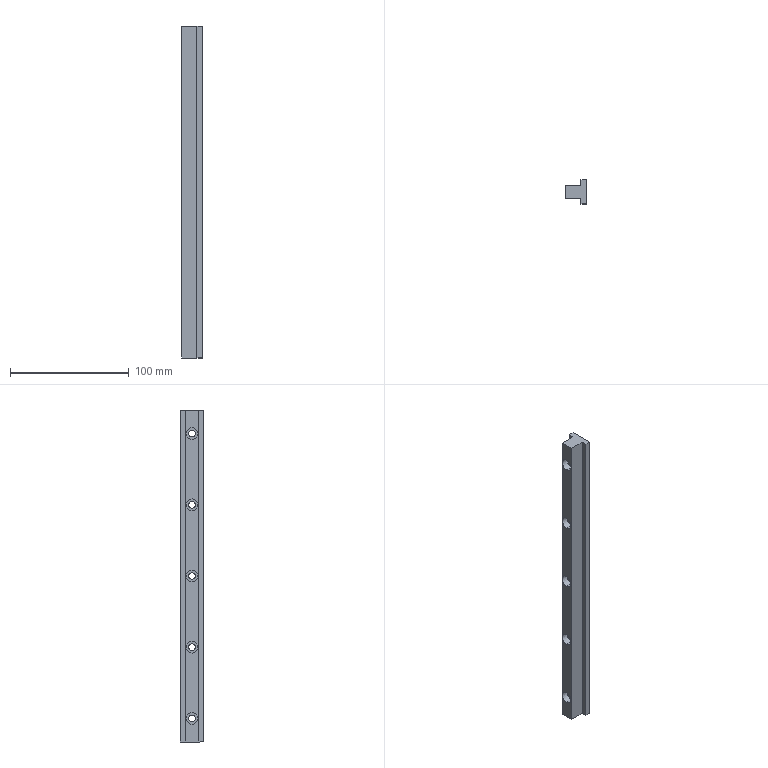Component | SolidWorks | GuideRailHGH-20CA-340-2 | 1 solid | 35 faces | box 17.5 x 20 x 280 mm | volume 61934 mm3 | cylinder 20 | plane 15 | commonest cylinder face diameters 5.5 x10 10 x10
build123d program:
from build123d import *

# Parameters (mm, degrees)
SKETCH1_W                                       = 20
SKETCH1_H                                       = 17.5
BOSS_EXTRUDE1_DEPTH                             = 280
SKETCH2_W                                       = 4.5
SKETCH2_H                                       = 12.9
CUT_EXTRUDE1_DEPTH                              = 280
M5_HEX_SOCKET_HEAD_CAP_SCREW_CBORE2_D           = 5.5
M5_HEX_SOCKET_HEAD_CAP_SCREW_CBORE2_CBORE_D     = 10
M5_HEX_SOCKET_HEAD_CAP_SCREW_CBORE2_CBORE_DEPTH = 5.4
LPATTERN1_COUNT                                 = 5
LPATTERN1_PITCH                                 = 60


with BuildPart() as part:
    # Sketch1 → Boss-Extrude1 (new body)
    with BuildSketch(Plane.XY):
        Rectangle(SKETCH1_W, SKETCH1_H)
    extrude(amount=BOSS_EXTRUDE1_DEPTH)

    # Sketch2 → Cut-Extrude1 (cut)
    with BuildSketch(Plane.XY.offset(280)):
        with Locations((-7.75, 2.3)):
            Rectangle(SKETCH2_W, SKETCH2_H)
        with Locations((7.75, 2.3)):
            Rectangle(SKETCH2_W, SKETCH2_H)
    extrude(amount=-CUT_EXTRUDE1_DEPTH, mode=Mode.SUBTRACT)

    # M5 Hex Socket Head Cap Screw CBORE2 (through all)
    with Locations(Plane(origin=(0, 8.75, 0), x_dir=(1, 0, 0), z_dir=(0, 1, 0))):
        with Locations((0, -260)):
            m5_hex_socket_head_cap_screw_cbore2 = CounterBoreHole(M5_HEX_SOCKET_HEAD_CAP_SCREW_CBORE2_D / 2, M5_HEX_SOCKET_HEAD_CAP_SCREW_CBORE2_CBORE_D / 2, M5_HEX_SOCKET_HEAD_CAP_SCREW_CBORE2_CBORE_DEPTH)

    # LPattern1: M5 Hex Socket Head Cap Screw CBORE2 ×5
    with Locations(*[(0, 0, -i * LPATTERN1_PITCH) for i in range(1, LPATTERN1_COUNT)]):
        add(m5_hex_socket_head_cap_screw_cbore2, mode=Mode.SUBTRACT)


solid = part.part

# Placed as in the assembly
solid = solid.moved(Location((1977.413, 3833.763, 939.241), (0, 0, 90)))
STEP:
#1=CARTESIAN_POINT('',(78.195,150.936,47.322));
#2=VERTEX_POINT('',#1);
#3=CARTESIAN_POINT('',(78.195,150.936,47.106));
#4=VERTEX_POINT('',#3);
#5=CARTESIAN_POINT('',(78.195,150.936,47.214));
#6=DIRECTION('',(-1.,-0.0001552,-0.));
#7=DIRECTION('',(0.,0.,-1.));
#8=AXIS2_PLACEMENT_3D('',#5,#6,#7);
#9=CIRCLE('',#8,0.1083);
#10=EDGE_CURVE('',#2,#4,#9,.T.);
#11=ORIENTED_EDGE('',*,*,#10,.F.);
#12=CARTESIAN_POINT('',(77.719,150.936,47.322));
#13=VERTEX_POINT('',#12);
#14=CARTESIAN_POINT('',(77.506,150.935,47.322));
#15=DIRECTION('',(-1.,-0.0001552,-0.));
#16=VECTOR('',#15,39.37);
#17=LINE('',#14,#16);
#18=EDGE_CURVE('',#2,#13,#17,.T.);
#19=ORIENTED_EDGE('',*,*,#18,.T.);
#20=CARTESIAN_POINT('',(77.719,150.936,47.106));
#21=VERTEX_POINT('',#20);
#22=CARTESIAN_POINT('',(77.719,150.936,47.214));
#23=DIRECTION('',(-1.,-0.0001552,-0.));
#24=DIRECTION('',(0.,0.,-1.));
#25=AXIS2_PLACEMENT_3D('',#22,#23,#24);
#26=CIRCLE('',#25,0.1083);
#27=EDGE_CURVE('',#13,#21,#26,.T.);
#28=ORIENTED_EDGE('',*,*,#27,.T.);
#29=CARTESIAN_POINT('',(77.506,150.935,47.106));
#30=DIRECTION('',(-1.,-0.0001552,-0.));
#31=VECTOR('',#30,39.37);
#32=LINE('',#29,#31);
#33=EDGE_CURVE('',#4,#21,#32,.T.);
#34=ORIENTED_EDGE('',*,*,#33,.F.);
#35=EDGE_LOOP('',(#11,#19,#28,#34));
#36=FACE_OUTER_BOUND('',#35,.T.);
#37=CARTESIAN_POINT('',(77.506,150.935,47.214));
#38=DIRECTION('',(-1.,-0.0001552,-0.));
#39=DIRECTION('',(0.,0.,-1.));
#40=AXIS2_PLACEMENT_3D('',#37,#38,#39);
#41=CYLINDRICAL_SURFACE('',#40,0.1083);
#42=ADVANCED_FACE('',(#36),#41,.F.);
#43=CARTESIAN_POINT('',(77.719,150.936,47.411));
#44=VERTEX_POINT('',#43);
#45=CARTESIAN_POINT('',(77.719,150.936,47.017));
#46=VERTEX_POINT('',#45);
#47=CARTESIAN_POINT('',(77.719,150.936,47.214));
#48=DIRECTION('',(-1.,-0.0001552,-0.));
#49=DIRECTION('',(0.,0.,-1.));
#50=AXIS2_PLACEMENT_3D('',#47,#48,#49);
#51=CIRCLE('',#50,0.1969);
#52=EDGE_CURVE('',#44,#46,#51,.T.);
#53=ORIENTED_EDGE('',*,*,#52,.F.);
#54=CARTESIAN_POINT('',(77.506,150.935,47.411));
#55=VERTEX_POINT('',#54);
#56=CARTESIAN_POINT('',(77.506,150.935,47.411));
#57=DIRECTION('',(-1.,-0.0001552,-0.));
#58=VECTOR('',#57,39.37);
#59=LINE('',#56,#58);
#60=EDGE_CURVE('',#44,#55,#59,.T.);
#61=ORIENTED_EDGE('',*,*,#60,.T.);
#62=CARTESIAN_POINT('',(77.506,150.935,47.017));
#63=VERTEX_POINT('',#62);
#64=CARTESIAN_POINT('',(77.506,150.935,47.214));
#65=DIRECTION('',(-1.,-0.0001552,-0.));
#66=DIRECTION('',(0.,0.,-1.));
#67=AXIS2_PLACEMENT_3D('',#64,#65,#66);
#68=CIRCLE('',#67,0.1969);
#69=EDGE_CURVE('',#55,#63,#68,.T.);
#70=ORIENTED_EDGE('',*,*,#69,.T.);
#71=CARTESIAN_POINT('',(77.506,150.935,47.017));
#72=DIRECTION('',(-1.,-0.0001552,-0.));
#73=VECTOR('',#72,39.37);
#74=LINE('',#71,#73);
#75=EDGE_CURVE('',#46,#63,#74,.T.);
#76=ORIENTED_EDGE('',*,*,#75,.F.);
#77=EDGE_LOOP('',(#53,#61,#70,#76));
#78=FACE_OUTER_BOUND('',#77,.T.);
#79=CARTESIAN_POINT('',(77.506,150.935,47.214));
#80=DIRECTION('',(-1.,-0.0001552,-0.));
#81=DIRECTION('',(0.,0.,-1.));
#82=AXIS2_PLACEMENT_3D('',#79,#80,#81);
#83=CYLINDRICAL_SURFACE('',#82,0.1969);
#84=ADVANCED_FACE('',(#78),#83,.F.);
#85=CARTESIAN_POINT('',(78.195,150.936,44.96));
#86=VERTEX_POINT('',#85);
#87=CARTESIAN_POINT('',(78.195,150.936,44.744));
#88=VERTEX_POINT('',#87);
#89=CARTESIAN_POINT('',(78.195,150.936,44.852));
#90=DIRECTION('',(-1.,-0.0001552,-0.));
#91=DIRECTION('',(0.,0.,-1.));
#92=AXIS2_PLACEMENT_3D('',#89,#90,#91);
#93=CIRCLE('',#92,0.1083);
#94=EDGE_CURVE('',#86,#88,#93,.T.);
#95=ORIENTED_EDGE('',*,*,#94,.F.);
#96=CARTESIAN_POINT('',(77.719,150.936,44.96));
#97=VERTEX_POINT('',#96);
#98=CARTESIAN_POINT('',(77.506,150.935,44.96));
#99=DIRECTION('',(-1.,-0.0001552,-0.));
#100=VECTOR('',#99,39.37);
#101=LINE('',#98,#100);
#102=EDGE_CURVE('',#86,#97,#101,.T.);
#103=ORIENTED_EDGE('',*,*,#102,.T.);
#104=CARTESIAN_POINT('',(77.719,150.936,44.744));
#105=VERTEX_POINT('',#104);
#106=CARTESIAN_POINT('',(77.719,150.936,44.852));
#107=DIRECTION('',(-1.,-0.0001552,-0.));
#108=DIRECTION('',(0.,0.,-1.));
#109=AXIS2_PLACEMENT_3D('',#106,#107,#108);
#110=CIRCLE('',#109,0.1083);
#111=EDGE_CURVE('',#97,#105,#110,.T.);
#112=ORIENTED_EDGE('',*,*,#111,.T.);
#113=CARTESIAN_POINT('',(77.506,150.935,44.744));
#114=DIRECTION('',(-1.,-0.0001552,-0.));
#115=VECTOR('',#114,39.37);
#116=LINE('',#113,#115);
#117=EDGE_CURVE('',#88,#105,#116,.T.);
#118=ORIENTED_EDGE('',*,*,#117,.F.);
#119=EDGE_LOOP('',(#95,#103,#112,#118));
#120=FACE_OUTER_BOUND('',#119,.T.);
#121=CARTESIAN_POINT('',(77.506,150.935,44.852));
#122=DIRECTION('',(-1.,-0.0001552,-0.));
#123=DIRECTION('',(0.,0.,-1.));
#124=AXIS2_PLACEMENT_3D('',#121,#122,#123);
#125=CYLINDRICAL_SURFACE('',#124,0.1083);
#126=ADVANCED_FACE('',(#120),#125,.F.);
#127=CARTESIAN_POINT('',(77.719,150.936,45.049));
#128=VERTEX_POINT('',#127);
#129=CARTESIAN_POINT('',(77.719,150.936,44.655));
#130=VERTEX_POINT('',#129);
#131=CARTESIAN_POINT('',(77.719,150.936,44.852));
#132=DIRECTION('',(-1.,-0.0001552,-0.));
#133=DIRECTION('',(0.,0.,-1.));
#134=AXIS2_PLACEMENT_3D('',#131,#132,#133);
#135=CIRCLE('',#134,0.1969);
#136=EDGE_CURVE('',#128,#130,#135,.T.);
#137=ORIENTED_EDGE('',*,*,#136,.F.);
#138=CARTESIAN_POINT('',(77.506,150.935,45.049));
#139=VERTEX_POINT('',#138);
#140=CARTESIAN_POINT('',(77.506,150.935,45.049));
#141=DIRECTION('',(-1.,-0.0001552,-0.));
#142=VECTOR('',#141,39.37);
#143=LINE('',#140,#142);
#144=EDGE_CURVE('',#128,#139,#143,.T.);
#145=ORIENTED_EDGE('',*,*,#144,.T.);
#146=CARTESIAN_POINT('',(77.506,150.935,44.655));
#147=VERTEX_POINT('',#146);
#148=CARTESIAN_POINT('',(77.506,150.935,44.852));
#149=DIRECTION('',(-1.,-0.0001552,-0.));
#150=DIRECTION('',(0.,0.,-1.));
#151=AXIS2_PLACEMENT_3D('',#148,#149,#150);
#152=CIRCLE('',#151,0.1969);
#153=EDGE_CURVE('',#139,#147,#152,.T.);
#154=ORIENTED_EDGE('',*,*,#153,.T.);
#155=CARTESIAN_POINT('',(77.506,150.935,44.655));
#156=DIRECTION('',(-1.,-0.0001552,-0.));
#157=VECTOR('',#156,39.37);
#158=LINE('',#155,#157);
#159=EDGE_CURVE('',#130,#147,#158,.T.);
#160=ORIENTED_EDGE('',*,*,#159,.F.);
#161=EDGE_LOOP('',(#137,#145,#154,#160));
#162=FACE_OUTER_BOUND('',#161,.T.);
#163=CARTESIAN_POINT('',(77.506,150.935,44.852));
#164=DIRECTION('',(-1.,-0.0001552,-0.));
#165=DIRECTION('',(0.,0.,-1.));
#166=AXIS2_PLACEMENT_3D('',#163,#164,#165);
#167=CYLINDRICAL_SURFACE('',#166,0.1969);
#168=ADVANCED_FACE('',(#162),#167,.F.);
#169=CARTESIAN_POINT('',(78.195,150.936,42.598));
#170=VERTEX_POINT('',#169);
#171=CARTESIAN_POINT('',(78.195,150.936,42.382));
#172=VERTEX_POINT('',#171);
#173=CARTESIAN_POINT('',(78.195,150.936,42.49));
#174=DIRECTION('',(-1.,-0.0001552,-0.));
#175=DIRECTION('',(0.,0.,-1.));
#176=AXIS2_PLACEMENT_3D('',#173,#174,#175);
#177=CIRCLE('',#176,0.1083);
#178=EDGE_CURVE('',#170,#172,#177,.T.);
#179=ORIENTED_EDGE('',*,*,#178,.F.);
#180=CARTESIAN_POINT('',(77.719,150.936,42.598));
#181=VERTEX_POINT('',#180);
#182=CARTESIAN_POINT('',(77.506,150.935,42.598));
#183=DIRECTION('',(-1.,-0.0001552,-0.));
#184=VECTOR('',#183,39.37);
#185=LINE('',#182,#184);
#186=EDGE_CURVE('',#170,#181,#185,.T.);
#187=ORIENTED_EDGE('',*,*,#186,.T.);
#188=CARTESIAN_POINT('',(77.719,150.936,42.382));
#189=VERTEX_POINT('',#188);
#190=CARTESIAN_POINT('',(77.719,150.936,42.49));
#191=DIRECTION('',(-1.,-0.0001552,-0.));
#192=DIRECTION('',(0.,0.,-1.));
#193=AXIS2_PLACEMENT_3D('',#190,#191,#192);
#194=CIRCLE('',#193,0.1083);
#195=EDGE_CURVE('',#181,#189,#194,.T.);
#196=ORIENTED_EDGE('',*,*,#195,.T.);
#197=CARTESIAN_POINT('',(77.506,150.935,42.382));
#198=DIRECTION('',(-1.,-0.0001552,-0.));
#199=VECTOR('',#198,39.37);
#200=LINE('',#197,#199);
#201=EDGE_CURVE('',#172,#189,#200,.T.);
#202=ORIENTED_EDGE('',*,*,#201,.F.);
#203=EDGE_LOOP('',(#179,#187,#196,#202));
#204=FACE_OUTER_BOUND('',#203,.T.);
#205=CARTESIAN_POINT('',(77.506,150.935,42.49));
#206=DIRECTION('',(-1.,-0.0001552,-0.));
#207=DIRECTION('',(0.,0.,-1.));
#208=AXIS2_PLACEMENT_3D('',#205,#206,#207);
#209=CYLINDRICAL_SURFACE('',#208,0.1083);
#210=ADVANCED_FACE('',(#204),#209,.F.);
#211=CARTESIAN_POINT('',(77.719,150.936,42.687));
#212=VERTEX_POINT('',#211);
#213=CARTESIAN_POINT('',(77.719,150.936,42.293));
#214=VERTEX_POINT('',#213);
#215=CARTESIAN_POINT('',(77.719,150.936,42.49));
#216=DIRECTION('',(-1.,-0.0001552,-0.));
#217=DIRECTION('',(0.,0.,-1.));
#218=AXIS2_PLACEMENT_3D('',#215,#216,#217);
#219=CIRCLE('',#218,0.1969);
#220=EDGE_CURVE('',#212,#214,#219,.T.);
#221=ORIENTED_EDGE('',*,*,#220,.F.);
#222=CARTESIAN_POINT('',(77.506,150.935,42.687));
#223=VERTEX_POINT('',#222);
#224=CARTESIAN_POINT('',(77.506,150.935,42.687));
#225=DIRECTION('',(-1.,-0.0001552,-0.));
#226=VECTOR('',#225,39.37);
#227=LINE('',#224,#226);
#228=EDGE_CURVE('',#212,#223,#227,.T.);
#229=ORIENTED_EDGE('',*,*,#228,.T.);
#230=CARTESIAN_POINT('',(77.506,150.935,42.293));
#231=VERTEX_POINT('',#230);
#232=CARTESIAN_POINT('',(77.506,150.935,42.49));
#233=DIRECTION('',(-1.,-0.0001552,-0.));
#234=DIRECTION('',(0.,0.,-1.));
#235=AXIS2_PLACEMENT_3D('',#232,#233,#234);
#236=CIRCLE('',#235,0.1969);
#237=EDGE_CURVE('',#223,#231,#236,.T.);
#238=ORIENTED_EDGE('',*,*,#237,.T.);
#239=CARTESIAN_POINT('',(77.506,150.935,42.293));
#240=DIRECTION('',(-1.,-0.0001552,-0.));
#241=VECTOR('',#240,39.37);
#242=LINE('',#239,#241);
#243=EDGE_CURVE('',#214,#231,#242,.T.);
#244=ORIENTED_EDGE('',*,*,#243,.F.);
#245=EDGE_LOOP('',(#221,#229,#238,#244));
#246=FACE_OUTER_BOUND('',#245,.T.);
#247=CARTESIAN_POINT('',(77.506,150.935,42.49));
#248=DIRECTION('',(-1.,-0.0001552,-0.));
#249=DIRECTION('',(0.,0.,-1.));
#250=AXIS2_PLACEMENT_3D('',#247,#248,#249);
#251=CYLINDRICAL_SURFACE('',#250,0.1969);
#252=ADVANCED_FACE('',(#246),#251,.F.);
#253=CARTESIAN_POINT('',(77.719,150.936,40.324));
#254=VERTEX_POINT('',#253);
#255=CARTESIAN_POINT('',(77.719,150.936,39.931));
#256=VERTEX_POINT('',#255);
#257=CARTESIAN_POINT('',(77.719,150.936,40.128));
#258=DIRECTION('',(-1.,-0.0001552,-0.));
#259=DIRECTION('',(0.,0.,-1.));
#260=AXIS2_PLACEMENT_3D('',#257,#258,#259);
#261=CIRCLE('',#260,0.1969);
#262=EDGE_CURVE('',#254,#256,#261,.T.);
#263=ORIENTED_EDGE('',*,*,#262,.F.);
#264=CARTESIAN_POINT('',(77.506,150.935,40.324));
#265=VERTEX_POINT('',#264);
#266=CARTESIAN_POINT('',(77.506,150.935,40.324));
#267=DIRECTION('',(-1.,-0.0001552,-0.));
#268=VECTOR('',#267,39.37);
#269=LINE('',#266,#268);
#270=EDGE_CURVE('',#254,#265,#269,.T.);
#271=ORIENTED_EDGE('',*,*,#270,.T.);
#272=CARTESIAN_POINT('',(77.506,150.935,39.931));
#273=VERTEX_POINT('',#272);
#274=CARTESIAN_POINT('',(77.506,150.935,40.128));
#275=DIRECTION('',(-1.,-0.0001552,-0.));
#276=DIRECTION('',(0.,0.,-1.));
#277=AXIS2_PLACEMENT_3D('',#274,#275,#276);
#278=CIRCLE('',#277,0.1969);
#279=EDGE_CURVE('',#265,#273,#278,.T.);
#280=ORIENTED_EDGE('',*,*,#279,.T.);
#281=CARTESIAN_POINT('',(77.506,150.935,39.931));
#282=DIRECTION('',(-1.,-0.0001552,-0.));
#283=VECTOR('',#282,39.37);
#284=LINE('',#281,#283);
#285=EDGE_CURVE('',#256,#273,#284,.T.);
#286=ORIENTED_EDGE('',*,*,#285,.F.);
#287=EDGE_LOOP('',(#263,#271,#280,#286));
#288=FACE_OUTER_BOUND('',#287,.T.);
#289=CARTESIAN_POINT('',(77.506,150.935,40.128));
#290=DIRECTION('',(-1.,-0.0001552,-0.));
#291=DIRECTION('',(0.,0.,-1.));
#292=AXIS2_PLACEMENT_3D('',#289,#290,#291);
#293=CYLINDRICAL_SURFACE('',#292,0.1969);
#294=ADVANCED_FACE('',(#288),#293,.F.);
#295=CARTESIAN_POINT('',(78.195,150.936,40.236));
#296=VERTEX_POINT('',#295);
#297=CARTESIAN_POINT('',(78.195,150.936,40.019));
#298=VERTEX_POINT('',#297);
#299=CARTESIAN_POINT('',(78.195,150.936,40.128));
#300=DIRECTION('',(-1.,-0.0001552,-0.));
#301=DIRECTION('',(0.,0.,-1.));
#302=AXIS2_PLACEMENT_3D('',#299,#300,#301);
#303=CIRCLE('',#302,0.1083);
#304=EDGE_CURVE('',#296,#298,#303,.T.);
#305=ORIENTED_EDGE('',*,*,#304,.F.);
#306=CARTESIAN_POINT('',(77.719,150.936,40.236));
#307=VERTEX_POINT('',#306);
#308=CARTESIAN_POINT('',(77.506,150.935,40.236));
#309=DIRECTION('',(-1.,-0.0001552,-0.));
#310=VECTOR('',#309,39.37);
#311=LINE('',#308,#310);
#312=EDGE_CURVE('',#296,#307,#311,.T.);
#313=ORIENTED_EDGE('',*,*,#312,.T.);
#314=CARTESIAN_POINT('',(77.719,150.936,40.019));
#315=VERTEX_POINT('',#314);
#316=CARTESIAN_POINT('',(77.719,150.936,40.128));
#317=DIRECTION('',(-1.,-0.0001552,-0.));
#318=DIRECTION('',(0.,0.,-1.));
#319=AXIS2_PLACEMENT_3D('',#316,#317,#318);
#320=CIRCLE('',#319,0.1083);
#321=EDGE_CURVE('',#307,#315,#320,.T.);
#322=ORIENTED_EDGE('',*,*,#321,.T.);
#323=CARTESIAN_POINT('',(77.506,150.935,40.019));
#324=DIRECTION('',(-1.,-0.0001552,-0.));
#325=VECTOR('',#324,39.37);
#326=LINE('',#323,#325);
#327=EDGE_CURVE('',#298,#315,#326,.T.);
#328=ORIENTED_EDGE('',*,*,#327,.F.);
#329=EDGE_LOOP('',(#305,#313,#322,#328));
#330=FACE_OUTER_BOUND('',#329,.T.);
#331=CARTESIAN_POINT('',(77.506,150.935,40.128));
#332=DIRECTION('',(-1.,-0.0001552,-0.));
#333=DIRECTION('',(0.,0.,-1.));
#334=AXIS2_PLACEMENT_3D('',#331,#332,#333);
#335=CYLINDRICAL_SURFACE('',#334,0.1083);
#336=ADVANCED_FACE('',(#330),#335,.F.);
#337=CARTESIAN_POINT('',(77.719,150.936,37.962));
#338=VERTEX_POINT('',#337);
#339=CARTESIAN_POINT('',(77.719,150.936,37.569));
#340=VERTEX_POINT('',#339);
#341=CARTESIAN_POINT('',(77.719,150.936,37.765));
#342=DIRECTION('',(-1.,-0.0001552,-0.));
#343=DIRECTION('',(0.,0.,-1.));
#344=AXIS2_PLACEMENT_3D('',#341,#342,#343);
#345=CIRCLE('',#344,0.1969);
#346=EDGE_CURVE('',#338,#340,#345,.T.);
#347=ORIENTED_EDGE('',*,*,#346,.F.);
#348=CARTESIAN_POINT('',(77.506,150.935,37.962));
#349=VERTEX_POINT('',#348);
#350=CARTESIAN_POINT('',(77.506,150.935,37.962));
#351=DIRECTION('',(-1.,-0.0001552,-0.));
#352=VECTOR('',#351,39.37);
#353=LINE('',#350,#352);
#354=EDGE_CURVE('',#338,#349,#353,.T.);
#355=ORIENTED_EDGE('',*,*,#354,.T.);
#356=CARTESIAN_POINT('',(77.506,150.935,37.569));
#357=VERTEX_POINT('',#356);
#358=CARTESIAN_POINT('',(77.506,150.935,37.765));
#359=DIRECTION('',(-1.,-0.0001552,-0.));
#360=DIRECTION('',(0.,0.,-1.));
#361=AXIS2_PLACEMENT_3D('',#358,#359,#360);
#362=CIRCLE('',#361,0.1969);
#363=EDGE_CURVE('',#349,#357,#362,.T.);
#364=ORIENTED_EDGE('',*,*,#363,.T.);
#365=CARTESIAN_POINT('',(77.506,150.935,37.569));
#366=DIRECTION('',(-1.,-0.0001552,-0.));
#367=VECTOR('',#366,39.37);
#368=LINE('',#365,#367);
#369=EDGE_CURVE('',#340,#357,#368,.T.);
#370=ORIENTED_EDGE('',*,*,#369,.F.);
#371=EDGE_LOOP('',(#347,#355,#364,#370));
#372=FACE_OUTER_BOUND('',#371,.T.);
#373=CARTESIAN_POINT('',(77.506,150.935,37.765));
#374=DIRECTION('',(-1.,-0.0001552,-0.));
#375=DIRECTION('',(0.,0.,-1.));
#376=AXIS2_PLACEMENT_3D('',#373,#374,#375);
#377=CYLINDRICAL_SURFACE('',#376,0.1969);
#378=ADVANCED_FACE('',(#372),#377,.F.);
#379=CARTESIAN_POINT('',(78.195,150.936,37.874));
#380=VERTEX_POINT('',#379);
#381=CARTESIAN_POINT('',(78.195,150.936,37.657));
#382=VERTEX_POINT('',#381);
#383=CARTESIAN_POINT('',(78.195,150.936,37.765));
#384=DIRECTION('',(-1.,-0.0001552,-0.));
#385=DIRECTION('',(0.,0.,-1.));
#386=AXIS2_PLACEMENT_3D('',#383,#384,#385);
#387=CIRCLE('',#386,0.1083);
#388=EDGE_CURVE('',#380,#382,#387,.T.);
#389=ORIENTED_EDGE('',*,*,#388,.F.);
#390=CARTESIAN_POINT('',(77.719,150.936,37.874));
#391=VERTEX_POINT('',#390);
#392=CARTESIAN_POINT('',(77.506,150.935,37.874));
#393=DIRECTION('',(-1.,-0.0001552,-0.));
#394=VECTOR('',#393,39.37);
#395=LINE('',#392,#394);
#396=EDGE_CURVE('',#380,#391,#395,.T.);
#397=ORIENTED_EDGE('',*,*,#396,.T.);
#398=CARTESIAN_POINT('',(77.719,150.936,37.657));
#399=VERTEX_POINT('',#398);
#400=CARTESIAN_POINT('',(77.719,150.936,37.765));
#401=DIRECTION('',(-1.,-0.0001552,-0.));
#402=DIRECTION('',(0.,0.,-1.));
#403=AXIS2_PLACEMENT_3D('',#400,#401,#402);
#404=CIRCLE('',#403,0.1083);
#405=EDGE_CURVE('',#391,#399,#404,.T.);
#406=ORIENTED_EDGE('',*,*,#405,.T.);
#407=CARTESIAN_POINT('',(77.506,150.935,37.657));
#408=DIRECTION('',(-1.,-0.0001552,-0.));
#409=VECTOR('',#408,39.37);
#410=LINE('',#407,#409);
#411=EDGE_CURVE('',#382,#399,#410,.T.);
#412=ORIENTED_EDGE('',*,*,#411,.F.);
#413=EDGE_LOOP('',(#389,#397,#406,#412));
#414=FACE_OUTER_BOUND('',#413,.T.);
#415=CARTESIAN_POINT('',(77.506,150.935,37.765));
#416=DIRECTION('',(-1.,-0.0001552,-0.));
#417=DIRECTION('',(0.,0.,-1.));
#418=AXIS2_PLACEMENT_3D('',#415,#416,#417);
#419=CYLINDRICAL_SURFACE('',#418,0.1083);
#420=ADVANCED_FACE('',(#414),#419,.F.);
#421=CARTESIAN_POINT('',(78.014,151.329,36.978));
#422=VERTEX_POINT('',#421);
#423=CARTESIAN_POINT('',(78.195,151.329,36.978));
#424=VERTEX_POINT('',#423);
#425=CARTESIAN_POINT('',(78.195,151.329,36.978));
#426=DIRECTION('',(1.,0.0001552,0.));
#427=VECTOR('',#426,39.37);
#428=LINE('',#425,#427);
#429=EDGE_CURVE('',#422,#424,#428,.T.);
#430=ORIENTED_EDGE('',*,*,#429,.F.);
#431=CARTESIAN_POINT('',(78.014,151.329,48.002));
#432=VERTEX_POINT('',#431);
#433=CARTESIAN_POINT('',(78.014,151.329,48.54));
#434=DIRECTION('',(0.,-0.,-1.));
#435=VECTOR('',#434,39.37);
#436=LINE('',#433,#435);
#437=EDGE_CURVE('',#432,#422,#436,.T.);
#438=ORIENTED_EDGE('',*,*,#437,.F.);
#439=CARTESIAN_POINT('',(78.195,151.329,48.002));
#440=VERTEX_POINT('',#439);
#441=CARTESIAN_POINT('',(78.195,151.329,48.002));
#442=DIRECTION('',(1.,0.0001552,0.));
#443=VECTOR('',#442,39.37);
#444=LINE('',#441,#443);
#445=EDGE_CURVE('',#432,#440,#444,.T.);
#446=ORIENTED_EDGE('',*,*,#445,.T.);
#447=CARTESIAN_POINT('',(78.195,151.329,36.978));
#448=DIRECTION('',(-0.,0.,1.));
#449=VECTOR('',#448,39.37);
#450=LINE('',#447,#449);
#451=EDGE_CURVE('',#424,#440,#450,.T.);
#452=ORIENTED_EDGE('',*,*,#451,.F.);
#453=EDGE_LOOP('',(#430,#438,#446,#452));
#454=FACE_OUTER_BOUND('',#453,.T.);
#455=CARTESIAN_POINT('',(78.195,151.329,36.978));
#456=DIRECTION('',(0.0001552,-1.,0.));
#457=DIRECTION('',(-0.,0.,1.));
#458=AXIS2_PLACEMENT_3D('',#455,#456,#457);
#459=PLANE('',#458);
#460=ADVANCED_FACE('',(#454),#459,.F.);
#461=CARTESIAN_POINT('',(78.195,150.936,40.128));
#462=DIRECTION('',(-1.,-0.0001552,-0.));
#463=DIRECTION('',(0.,0.,-1.));
#464=AXIS2_PLACEMENT_3D('',#461,#462,#463);
#465=CIRCLE('',#464,0.1083);
#466=EDGE_CURVE('',#298,#296,#465,.T.);
#467=ORIENTED_EDGE('',*,*,#466,.T.);
#468=ORIENTED_EDGE('',*,*,#304,.T.);
#469=EDGE_LOOP('',(#467,#468));
#470=FACE_BOUND('',#469,.T.);
#471=CARTESIAN_POINT('',(78.195,150.936,37.765));
#472=DIRECTION('',(-1.,-0.0001552,-0.));
#473=DIRECTION('',(0.,0.,-1.));
#474=AXIS2_PLACEMENT_3D('',#471,#472,#473);
#475=CIRCLE('',#474,0.1083);
#476=EDGE_CURVE('',#382,#380,#475,.T.);
#477=ORIENTED_EDGE('',*,*,#476,.T.);
#478=ORIENTED_EDGE('',*,*,#388,.T.);
#479=EDGE_LOOP('',(#477,#478));
#480=FACE_BOUND('',#479,.T.);
#481=CARTESIAN_POINT('',(78.195,150.542,48.002));
#482=VERTEX_POINT('',#481);
#483=CARTESIAN_POINT('',(78.195,150.542,48.002));
#484=DIRECTION('',(0.0001552,-1.,0.));
#485=VECTOR('',#484,39.37);
#486=LINE('',#483,#485);
#487=EDGE_CURVE('',#440,#482,#486,.T.);
#488=ORIENTED_EDGE('',*,*,#487,.T.);
#489=CARTESIAN_POINT('',(78.195,150.542,36.978));
#490=VERTEX_POINT('',#489);
#491=CARTESIAN_POINT('',(78.195,150.542,36.978));
#492=DIRECTION('',(-0.,0.,1.));
#493=VECTOR('',#492,39.37);
#494=LINE('',#491,#493);
#495=EDGE_CURVE('',#490,#482,#494,.T.);
#496=ORIENTED_EDGE('',*,*,#495,.F.);
#497=CARTESIAN_POINT('',(78.195,150.542,36.978));
#498=DIRECTION('',(0.0001552,-1.,0.));
#499=VECTOR('',#498,39.37);
#500=LINE('',#497,#499);
#501=EDGE_CURVE('',#424,#490,#500,.T.);
#502=ORIENTED_EDGE('',*,*,#501,.F.);
#503=ORIENTED_EDGE('',*,*,#451,.T.);
#504=EDGE_LOOP('',(#488,#496,#502,#503));
#505=FACE_OUTER_BOUND('',#504,.T.);
#506=CARTESIAN_POINT('',(78.195,150.936,42.49));
#507=DIRECTION('',(-1.,-0.0001552,-0.));
#508=DIRECTION('',(0.,0.,-1.));
#509=AXIS2_PLACEMENT_3D('',#506,#507,#508);
#510=CIRCLE('',#509,0.1083);
#511=EDGE_CURVE('',#172,#170,#510,.T.);
#512=ORIENTED_EDGE('',*,*,#511,.T.);
#513=ORIENTED_EDGE('',*,*,#178,.T.);
#514=EDGE_LOOP('',(#512,#513));
#515=FACE_BOUND('',#514,.T.);
#516=CARTESIAN_POINT('',(78.195,150.936,44.852));
#517=DIRECTION('',(-1.,-0.0001552,-0.));
#518=DIRECTION('',(0.,0.,-1.));
#519=AXIS2_PLACEMENT_3D('',#516,#517,#518);
#520=CIRCLE('',#519,0.1083);
#521=EDGE_CURVE('',#88,#86,#520,.T.);
#522=ORIENTED_EDGE('',*,*,#521,.T.);
#523=ORIENTED_EDGE('',*,*,#94,.T.);
#524=EDGE_LOOP('',(#522,#523));
#525=FACE_BOUND('',#524,.T.);
#526=CARTESIAN_POINT('',(78.195,150.936,47.214));
#527=DIRECTION('',(-1.,-0.0001552,-0.));
#528=DIRECTION('',(0.,0.,-1.));
#529=AXIS2_PLACEMENT_3D('',#526,#527,#528);
#530=CIRCLE('',#529,0.1083);
#531=EDGE_CURVE('',#4,#2,#530,.T.);
#532=ORIENTED_EDGE('',*,*,#531,.T.);
#533=ORIENTED_EDGE('',*,*,#10,.T.);
#534=EDGE_LOOP('',(#532,#533));
#535=FACE_BOUND('',#534,.T.);
#536=CARTESIAN_POINT('',(78.195,150.542,36.978));
#537=DIRECTION('',(-1.,-0.0001552,-0.));
#538=DIRECTION('',(-0.0001552,1.,-0.));
#539=AXIS2_PLACEMENT_3D('',#536,#537,#538);
#540=PLANE('',#539);
#541=ADVANCED_FACE('',(#470,#480,#505,#515,#525,#535),#540,.F.);
#542=CARTESIAN_POINT('',(78.014,150.542,48.002));
#543=VERTEX_POINT('',#542);
#544=CARTESIAN_POINT('',(78.195,150.542,48.002));
#545=DIRECTION('',(-1.,-0.0001552,-0.));
#546=VECTOR('',#545,39.37);
#547=LINE('',#544,#546);
#548=EDGE_CURVE('',#482,#543,#547,.T.);
#549=ORIENTED_EDGE('',*,*,#548,.T.);
#550=CARTESIAN_POINT('',(78.014,150.542,36.978));
#551=VERTEX_POINT('',#550);
#552=CARTESIAN_POINT('',(78.014,150.542,48.54));
#553=DIRECTION('',(0.,-0.,-1.));
#554=VECTOR('',#553,39.37);
#555=LINE('',#552,#554);
#556=EDGE_CURVE('',#543,#551,#555,.T.);
#557=ORIENTED_EDGE('',*,*,#556,.T.);
#558=CARTESIAN_POINT('',(78.195,150.542,36.978));
#559=DIRECTION('',(-1.,-0.0001552,-0.));
#560=VECTOR('',#559,39.37);
#561=LINE('',#558,#560);
#562=EDGE_CURVE('',#490,#551,#561,.T.);
#563=ORIENTED_EDGE('',*,*,#562,.F.);
#564=ORIENTED_EDGE('',*,*,#495,.T.);
#565=EDGE_LOOP('',(#549,#557,#563,#564));
#566=FACE_OUTER_BOUND('',#565,.T.);
#567=CARTESIAN_POINT('',(78.195,150.542,36.978));
#568=DIRECTION('',(-0.0001552,1.,-0.));
#569=DIRECTION('',(0.,-0.,-1.));
#570=AXIS2_PLACEMENT_3D('',#567,#568,#569);
#571=PLANE('',#570);
#572=ADVANCED_FACE('',(#566),#571,.F.);
#573=CARTESIAN_POINT('',(77.506,150.935,40.128));
#574=DIRECTION('',(-1.,-0.0001552,-0.));
#575=DIRECTION('',(0.,0.,-1.));
#576=AXIS2_PLACEMENT_3D('',#573,#574,#575);
#577=CIRCLE('',#576,0.1969);
#578=EDGE_CURVE('',#273,#265,#577,.T.);
#579=ORIENTED_EDGE('',*,*,#578,.F.);
#580=ORIENTED_EDGE('',*,*,#279,.F.);
#581=EDGE_LOOP('',(#579,#580));
#582=FACE_BOUND('',#581,.T.);
#583=CARTESIAN_POINT('',(77.506,150.935,37.765));
#584=DIRECTION('',(-1.,-0.0001552,-0.));
#585=DIRECTION('',(0.,0.,-1.));
#586=AXIS2_PLACEMENT_3D('',#583,#584,#585);
#587=CIRCLE('',#586,0.1969);
#588=EDGE_CURVE('',#357,#349,#587,.T.);
#589=ORIENTED_EDGE('',*,*,#588,.F.);
#590=ORIENTED_EDGE('',*,*,#363,.F.);
#591=EDGE_LOOP('',(#589,#590));
#592=FACE_BOUND('',#591,.T.);
#593=CARTESIAN_POINT('',(77.506,150.719,36.978));
#594=VERTEX_POINT('',#593);
#595=CARTESIAN_POINT('',(77.506,151.152,36.978));
#596=VERTEX_POINT('',#595);
#597=CARTESIAN_POINT('',(77.506,150.542,36.978));
#598=DIRECTION('',(-0.0001552,1.,-0.));
#599=VECTOR('',#598,39.37);
#600=LINE('',#597,#599);
#601=EDGE_CURVE('',#594,#596,#600,.T.);
#602=ORIENTED_EDGE('',*,*,#601,.F.);
#603=CARTESIAN_POINT('',(77.506,150.719,48.002));
#604=VERTEX_POINT('',#603);
#605=CARTESIAN_POINT('',(77.506,150.719,48.54));
#606=DIRECTION('',(0.,-0.,-1.));
#607=VECTOR('',#606,39.37);
#608=LINE('',#605,#607);
#609=EDGE_CURVE('',#604,#594,#608,.T.);
#610=ORIENTED_EDGE('',*,*,#609,.F.);
#611=CARTESIAN_POINT('',(77.506,151.152,48.002));
#612=VERTEX_POINT('',#611);
#613=CARTESIAN_POINT('',(77.506,150.542,48.002));
#614=DIRECTION('',(-0.0001552,1.,-0.));
#615=VECTOR('',#614,39.37);
#616=LINE('',#613,#615);
#617=EDGE_CURVE('',#604,#612,#616,.T.);
#618=ORIENTED_EDGE('',*,*,#617,.T.);
#619=CARTESIAN_POINT('',(77.506,151.152,48.54));
#620=DIRECTION('',(0.,-0.,-1.));
#621=VECTOR('',#620,39.37);
#622=LINE('',#619,#621);
#623=EDGE_CURVE('',#612,#596,#622,.T.);
#624=ORIENTED_EDGE('',*,*,#623,.T.);
#625=EDGE_LOOP('',(#602,#610,#618,#624));
#626=FACE_OUTER_BOUND('',#625,.T.);
#627=CARTESIAN_POINT('',(77.506,150.935,42.49));
#628=DIRECTION('',(-1.,-0.0001552,-0.));
#629=DIRECTION('',(0.,0.,-1.));
#630=AXIS2_PLACEMENT_3D('',#627,#628,#629);
#631=CIRCLE('',#630,0.1969);
#632=EDGE_CURVE('',#231,#223,#631,.T.);
#633=ORIENTED_EDGE('',*,*,#632,.F.);
#634=ORIENTED_EDGE('',*,*,#237,.F.);
#635=EDGE_LOOP('',(#633,#634));
#636=FACE_BOUND('',#635,.T.);
#637=CARTESIAN_POINT('',(77.506,150.935,44.852));
#638=DIRECTION('',(-1.,-0.0001552,-0.));
#639=DIRECTION('',(0.,0.,-1.));
#640=AXIS2_PLACEMENT_3D('',#637,#638,#639);
#641=CIRCLE('',#640,0.1969);
#642=EDGE_CURVE('',#147,#139,#641,.T.);
#643=ORIENTED_EDGE('',*,*,#642,.F.);
#644=ORIENTED_EDGE('',*,*,#153,.F.);
#645=EDGE_LOOP('',(#643,#644));
#646=FACE_BOUND('',#645,.T.);
#647=CARTESIAN_POINT('',(77.506,150.935,47.214));
#648=DIRECTION('',(-1.,-0.0001552,-0.));
#649=DIRECTION('',(0.,0.,-1.));
#650=AXIS2_PLACEMENT_3D('',#647,#648,#649);
#651=CIRCLE('',#650,0.1969);
#652=EDGE_CURVE('',#63,#55,#651,.T.);
#653=ORIENTED_EDGE('',*,*,#652,.F.);
#654=ORIENTED_EDGE('',*,*,#69,.F.);
#655=EDGE_LOOP('',(#653,#654));
#656=FACE_BOUND('',#655,.T.);
#657=CARTESIAN_POINT('',(77.506,150.542,36.978));
#658=DIRECTION('',(1.,0.0001552,0.));
#659=DIRECTION('',(0.0001552,-1.,0.));
#660=AXIS2_PLACEMENT_3D('',#657,#658,#659);
#661=PLANE('',#660);
#662=ADVANCED_FACE('',(#582,#592,#626,#636,#646,#656),#661,.F.);
#663=CARTESIAN_POINT('',(78.014,150.719,36.978));
#664=VERTEX_POINT('',#663);
#665=CARTESIAN_POINT('',(78.014,150.542,36.978));
#666=DIRECTION('',(0.0001552,-1.,0.));
#667=VECTOR('',#666,39.37);
#668=LINE('',#665,#667);
#669=EDGE_CURVE('',#664,#551,#668,.T.);
#670=ORIENTED_EDGE('',*,*,#669,.F.);
#671=CARTESIAN_POINT('',(78.014,150.719,36.978));
#672=DIRECTION('',(1.,0.0001552,0.));
#673=VECTOR('',#672,39.37);
#674=LINE('',#671,#673);
#675=EDGE_CURVE('',#594,#664,#674,.T.);
#676=ORIENTED_EDGE('',*,*,#675,.F.);
#677=ORIENTED_EDGE('',*,*,#601,.T.);
#678=CARTESIAN_POINT('',(78.014,151.152,36.978));
#679=VERTEX_POINT('',#678);
#680=CARTESIAN_POINT('',(78.014,151.152,36.978));
#681=DIRECTION('',(-1.,-0.0001552,-0.));
#682=VECTOR('',#681,39.37);
#683=LINE('',#680,#682);
#684=EDGE_CURVE('',#679,#596,#683,.T.);
#685=ORIENTED_EDGE('',*,*,#684,.F.);
#686=CARTESIAN_POINT('',(78.014,151.329,36.978));
#687=DIRECTION('',(0.0001552,-1.,0.));
#688=VECTOR('',#687,39.37);
#689=LINE('',#686,#688);
#690=EDGE_CURVE('',#422,#679,#689,.T.);
#691=ORIENTED_EDGE('',*,*,#690,.F.);
#692=ORIENTED_EDGE('',*,*,#429,.T.);
#693=ORIENTED_EDGE('',*,*,#501,.T.);
#694=ORIENTED_EDGE('',*,*,#562,.T.);
#695=EDGE_LOOP('',(#670,#676,#677,#685,#691,#692,#693,#694));
#696=FACE_OUTER_BOUND('',#695,.T.);
#697=CARTESIAN_POINT('',(77.851,150.936,36.978));
#698=DIRECTION('',(0.,-0.,-1.));
#699=DIRECTION('',(0.0001552,-1.,0.));
#700=AXIS2_PLACEMENT_3D('',#697,#698,#699);
#701=PLANE('',#700);
#702=ADVANCED_FACE('',(#696),#701,.T.);
#703=CARTESIAN_POINT('',(78.014,150.719,48.002));
#704=VERTEX_POINT('',#703);
#705=CARTESIAN_POINT('',(78.014,150.719,48.002));
#706=DIRECTION('',(-1.,-0.0001552,-0.));
#707=VECTOR('',#706,39.37);
#708=LINE('',#705,#707);
#709=EDGE_CURVE('',#704,#604,#708,.T.);
#710=ORIENTED_EDGE('',*,*,#709,.F.);
#711=CARTESIAN_POINT('',(78.014,150.542,48.002));
#712=DIRECTION('',(-0.0001552,1.,-0.));
#713=VECTOR('',#712,39.37);
#714=LINE('',#711,#713);
#715=EDGE_CURVE('',#543,#704,#714,.T.);
#716=ORIENTED_EDGE('',*,*,#715,.F.);
#717=ORIENTED_EDGE('',*,*,#548,.F.);
#718=ORIENTED_EDGE('',*,*,#487,.F.);
#719=ORIENTED_EDGE('',*,*,#445,.F.);
#720=CARTESIAN_POINT('',(78.014,151.152,48.002));
#721=VERTEX_POINT('',#720);
#722=CARTESIAN_POINT('',(78.014,151.329,48.002));
#723=DIRECTION('',(-0.0001552,1.,-0.));
#724=VECTOR('',#723,39.37);
#725=LINE('',#722,#724);
#726=EDGE_CURVE('',#721,#432,#725,.T.);
#727=ORIENTED_EDGE('',*,*,#726,.F.);
#728=CARTESIAN_POINT('',(78.014,151.152,48.002));
#729=DIRECTION('',(1.,0.0001552,0.));
#730=VECTOR('',#729,39.37);
#731=LINE('',#728,#730);
#732=EDGE_CURVE('',#612,#721,#731,.T.);
#733=ORIENTED_EDGE('',*,*,#732,.F.);
#734=ORIENTED_EDGE('',*,*,#617,.F.);
#735=EDGE_LOOP('',(#710,#716,#717,#718,#719,#727,#733,#734));
#736=FACE_OUTER_BOUND('',#735,.T.);
#737=CARTESIAN_POINT('',(77.851,150.936,48.002));
#738=DIRECTION('',(0.,-0.,-1.));
#739=DIRECTION('',(0.0001552,-1.,0.));
#740=AXIS2_PLACEMENT_3D('',#737,#738,#739);
#741=PLANE('',#740);
#742=ADVANCED_FACE('',(#736),#741,.F.);
#743=ORIENTED_EDGE('',*,*,#732,.T.);
#744=CARTESIAN_POINT('',(78.014,151.152,48.54));
#745=DIRECTION('',(0.,-0.,-1.));
#746=VECTOR('',#745,39.37);
#747=LINE('',#744,#746);
#748=EDGE_CURVE('',#721,#679,#747,.T.);
#749=ORIENTED_EDGE('',*,*,#748,.T.);
#750=ORIENTED_EDGE('',*,*,#684,.T.);
#751=ORIENTED_EDGE('',*,*,#623,.F.);
#752=EDGE_LOOP('',(#743,#749,#750,#751));
#753=FACE_OUTER_BOUND('',#752,.T.);
#754=CARTESIAN_POINT('',(78.014,151.152,48.54));
#755=DIRECTION('',(0.0001552,-1.,0.));
#756=DIRECTION('',(-0.,0.,1.));
#757=AXIS2_PLACEMENT_3D('',#754,#755,#756);
#758=PLANE('',#757);
#759=ADVANCED_FACE('',(#753),#758,.F.);
#760=ORIENTED_EDGE('',*,*,#726,.T.);
#761=ORIENTED_EDGE('',*,*,#437,.T.);
#762=ORIENTED_EDGE('',*,*,#690,.T.);
#763=ORIENTED_EDGE('',*,*,#748,.F.);
#764=EDGE_LOOP('',(#760,#761,#762,#763));
#765=FACE_OUTER_BOUND('',#764,.T.);
#766=CARTESIAN_POINT('',(78.014,151.329,48.54));
#767=DIRECTION('',(1.,0.0001552,0.));
#768=DIRECTION('',(-0.,0.,1.));
#769=AXIS2_PLACEMENT_3D('',#766,#767,#768);
#770=PLANE('',#769);
#771=ADVANCED_FACE('',(#765),#770,.F.);
#772=ORIENTED_EDGE('',*,*,#715,.T.);
#773=CARTESIAN_POINT('',(78.014,150.719,48.54));
#774=DIRECTION('',(0.,-0.,-1.));
#775=VECTOR('',#774,39.37);
#776=LINE('',#773,#775);
#777=EDGE_CURVE('',#704,#664,#776,.T.);
#778=ORIENTED_EDGE('',*,*,#777,.T.);
#779=ORIENTED_EDGE('',*,*,#669,.T.);
#780=ORIENTED_EDGE('',*,*,#556,.F.);
#781=EDGE_LOOP('',(#772,#778,#779,#780));
#782=FACE_OUTER_BOUND('',#781,.T.);
#783=CARTESIAN_POINT('',(78.014,150.542,48.54));
#784=DIRECTION('',(1.,0.0001552,0.));
#785=DIRECTION('',(-0.,0.,1.));
#786=AXIS2_PLACEMENT_3D('',#783,#784,#785);
#787=PLANE('',#786);
#788=ADVANCED_FACE('',(#782),#787,.F.);
#789=ORIENTED_EDGE('',*,*,#709,.T.);
#790=ORIENTED_EDGE('',*,*,#609,.T.);
#791=ORIENTED_EDGE('',*,*,#675,.T.);
#792=ORIENTED_EDGE('',*,*,#777,.F.);
#793=EDGE_LOOP('',(#789,#790,#791,#792));
#794=FACE_OUTER_BOUND('',#793,.T.);
#795=CARTESIAN_POINT('',(78.014,150.719,48.54));
#796=DIRECTION('',(-0.0001552,1.,-0.));
#797=DIRECTION('',(0.,-0.,-1.));
#798=AXIS2_PLACEMENT_3D('',#795,#796,#797);
#799=PLANE('',#798);
#800=ADVANCED_FACE('',(#794),#799,.F.);
#801=ORIENTED_EDGE('',*,*,#396,.F.);
#802=ORIENTED_EDGE('',*,*,#476,.F.);
#803=ORIENTED_EDGE('',*,*,#411,.T.);
#804=CARTESIAN_POINT('',(77.719,150.936,37.765));
#805=DIRECTION('',(-1.,-0.0001552,-0.));
#806=DIRECTION('',(0.,0.,-1.));
#807=AXIS2_PLACEMENT_3D('',#804,#805,#806);
#808=CIRCLE('',#807,0.1083);
#809=EDGE_CURVE('',#399,#391,#808,.T.);
#810=ORIENTED_EDGE('',*,*,#809,.T.);
#811=EDGE_LOOP('',(#801,#802,#803,#810));
#812=FACE_OUTER_BOUND('',#811,.T.);
#813=CARTESIAN_POINT('',(77.506,150.935,37.765));
#814=DIRECTION('',(-1.,-0.0001552,-0.));
#815=DIRECTION('',(0.,0.,-1.));
#816=AXIS2_PLACEMENT_3D('',#813,#814,#815);
#817=CYLINDRICAL_SURFACE('',#816,0.1083);
#818=ADVANCED_FACE('',(#812),#817,.F.);
#819=ORIENTED_EDGE('',*,*,#809,.F.);
#820=ORIENTED_EDGE('',*,*,#405,.F.);
#821=EDGE_LOOP('',(#819,#820));
#822=FACE_BOUND('',#821,.T.);
#823=CARTESIAN_POINT('',(77.719,150.936,37.765));
#824=DIRECTION('',(-1.,-0.0001552,-0.));
#825=DIRECTION('',(0.,0.,-1.));
#826=AXIS2_PLACEMENT_3D('',#823,#824,#825);
#827=CIRCLE('',#826,0.1969);
#828=EDGE_CURVE('',#340,#338,#827,.T.);
#829=ORIENTED_EDGE('',*,*,#828,.T.);
#830=ORIENTED_EDGE('',*,*,#346,.T.);
#831=EDGE_LOOP('',(#829,#830));
#832=FACE_OUTER_BOUND('',#831,.T.);
#833=CARTESIAN_POINT('',(77.719,150.827,37.765));
#834=DIRECTION('',(1.,0.0001552,0.));
#835=DIRECTION('',(-0.,0.,1.));
#836=AXIS2_PLACEMENT_3D('',#833,#834,#835);
#837=PLANE('',#836);
#838=ADVANCED_FACE('',(#822,#832),#837,.F.);
#839=ORIENTED_EDGE('',*,*,#354,.F.);
#840=ORIENTED_EDGE('',*,*,#828,.F.);
#841=ORIENTED_EDGE('',*,*,#369,.T.);
#842=ORIENTED_EDGE('',*,*,#588,.T.);
#843=EDGE_LOOP('',(#839,#840,#841,#842));
#844=FACE_OUTER_BOUND('',#843,.T.);
#845=CARTESIAN_POINT('',(77.506,150.935,37.765));
#846=DIRECTION('',(-1.,-0.0001552,-0.));
#847=DIRECTION('',(0.,0.,-1.));
#848=AXIS2_PLACEMENT_3D('',#845,#846,#847);
#849=CYLINDRICAL_SURFACE('',#848,0.1969);
#850=ADVANCED_FACE('',(#844),#849,.F.);
#851=ORIENTED_EDGE('',*,*,#312,.F.);
#852=ORIENTED_EDGE('',*,*,#466,.F.);
#853=ORIENTED_EDGE('',*,*,#327,.T.);
#854=CARTESIAN_POINT('',(77.719,150.936,40.128));
#855=DIRECTION('',(-1.,-0.0001552,-0.));
#856=DIRECTION('',(0.,0.,-1.));
#857=AXIS2_PLACEMENT_3D('',#854,#855,#856);
#858=CIRCLE('',#857,0.1083);
#859=EDGE_CURVE('',#315,#307,#858,.T.);
#860=ORIENTED_EDGE('',*,*,#859,.T.);
#861=EDGE_LOOP('',(#851,#852,#853,#860));
#862=FACE_OUTER_BOUND('',#861,.T.);
#863=CARTESIAN_POINT('',(77.506,150.935,40.128));
#864=DIRECTION('',(-1.,-0.0001552,-0.));
#865=DIRECTION('',(0.,0.,-1.));
#866=AXIS2_PLACEMENT_3D('',#863,#864,#865);
#867=CYLINDRICAL_SURFACE('',#866,0.1083);
#868=ADVANCED_FACE('',(#862),#867,.F.);
#869=ORIENTED_EDGE('',*,*,#859,.F.);
#870=ORIENTED_EDGE('',*,*,#321,.F.);
#871=EDGE_LOOP('',(#869,#870));
#872=FACE_BOUND('',#871,.T.);
#873=CARTESIAN_POINT('',(77.719,150.936,40.128));
#874=DIRECTION('',(-1.,-0.0001552,-0.));
#875=DIRECTION('',(0.,0.,-1.));
#876=AXIS2_PLACEMENT_3D('',#873,#874,#875);
#877=CIRCLE('',#876,0.1969);
#878=EDGE_CURVE('',#256,#254,#877,.T.);
#879=ORIENTED_EDGE('',*,*,#878,.T.);
#880=ORIENTED_EDGE('',*,*,#262,.T.);
#881=EDGE_LOOP('',(#879,#880));
#882=FACE_OUTER_BOUND('',#881,.T.);
#883=CARTESIAN_POINT('',(77.719,150.827,40.128));
#884=DIRECTION('',(1.,0.0001552,0.));
#885=DIRECTION('',(-0.,0.,1.));
#886=AXIS2_PLACEMENT_3D('',#883,#884,#885);
#887=PLANE('',#886);
#888=ADVANCED_FACE('',(#872,#882),#887,.F.);
#889=ORIENTED_EDGE('',*,*,#270,.F.);
#890=ORIENTED_EDGE('',*,*,#878,.F.);
#891=ORIENTED_EDGE('',*,*,#285,.T.);
#892=ORIENTED_EDGE('',*,*,#578,.T.);
#893=EDGE_LOOP('',(#889,#890,#891,#892));
#894=FACE_OUTER_BOUND('',#893,.T.);
#895=CARTESIAN_POINT('',(77.506,150.935,40.128));
#896=DIRECTION('',(-1.,-0.0001552,-0.));
#897=DIRECTION('',(0.,0.,-1.));
#898=AXIS2_PLACEMENT_3D('',#895,#896,#897);
#899=CYLINDRICAL_SURFACE('',#898,0.1969);
#900=ADVANCED_FACE('',(#894),#899,.F.);
#901=ORIENTED_EDGE('',*,*,#228,.F.);
#902=CARTESIAN_POINT('',(77.719,150.936,42.49));
#903=DIRECTION('',(-1.,-0.0001552,-0.));
#904=DIRECTION('',(0.,0.,-1.));
#905=AXIS2_PLACEMENT_3D('',#902,#903,#904);
#906=CIRCLE('',#905,0.1969);
#907=EDGE_CURVE('',#214,#212,#906,.T.);
#908=ORIENTED_EDGE('',*,*,#907,.F.);
#909=ORIENTED_EDGE('',*,*,#243,.T.);
#910=ORIENTED_EDGE('',*,*,#632,.T.);
#911=EDGE_LOOP('',(#901,#908,#909,#910));
#912=FACE_OUTER_BOUND('',#911,.T.);
#913=CARTESIAN_POINT('',(77.506,150.935,42.49));
#914=DIRECTION('',(-1.,-0.0001552,-0.));
#915=DIRECTION('',(0.,0.,-1.));
#916=AXIS2_PLACEMENT_3D('',#913,#914,#915);
#917=CYLINDRICAL_SURFACE('',#916,0.1969);
#918=ADVANCED_FACE('',(#912),#917,.F.);
#919=CARTESIAN_POINT('',(77.719,150.936,42.49));
#920=DIRECTION('',(-1.,-0.0001552,-0.));
#921=DIRECTION('',(0.,0.,-1.));
#922=AXIS2_PLACEMENT_3D('',#919,#920,#921);
#923=CIRCLE('',#922,0.1083);
#924=EDGE_CURVE('',#189,#181,#923,.T.);
#925=ORIENTED_EDGE('',*,*,#924,.F.);
#926=ORIENTED_EDGE('',*,*,#195,.F.);
#927=EDGE_LOOP('',(#925,#926));
#928=FACE_BOUND('',#927,.T.);
#929=ORIENTED_EDGE('',*,*,#907,.T.);
#930=ORIENTED_EDGE('',*,*,#220,.T.);
#931=EDGE_LOOP('',(#929,#930));
#932=FACE_OUTER_BOUND('',#931,.T.);
#933=CARTESIAN_POINT('',(77.719,150.827,42.49));
#934=DIRECTION('',(1.,0.0001552,0.));
#935=DIRECTION('',(-0.,0.,1.));
#936=AXIS2_PLACEMENT_3D('',#933,#934,#935);
#937=PLANE('',#936);
#938=ADVANCED_FACE('',(#928,#932),#937,.F.);
#939=ORIENTED_EDGE('',*,*,#186,.F.);
#940=ORIENTED_EDGE('',*,*,#511,.F.);
#941=ORIENTED_EDGE('',*,*,#201,.T.);
#942=ORIENTED_EDGE('',*,*,#924,.T.);
#943=EDGE_LOOP('',(#939,#940,#941,#942));
#944=FACE_OUTER_BOUND('',#943,.T.);
#945=CARTESIAN_POINT('',(77.506,150.935,42.49));
#946=DIRECTION('',(-1.,-0.0001552,-0.));
#947=DIRECTION('',(0.,0.,-1.));
#948=AXIS2_PLACEMENT_3D('',#945,#946,#947);
#949=CYLINDRICAL_SURFACE('',#948,0.1083);
#950=ADVANCED_FACE('',(#944),#949,.F.);
#951=ORIENTED_EDGE('',*,*,#144,.F.);
#952=CARTESIAN_POINT('',(77.719,150.936,44.852));
#953=DIRECTION('',(-1.,-0.0001552,-0.));
#954=DIRECTION('',(0.,0.,-1.));
#955=AXIS2_PLACEMENT_3D('',#952,#953,#954);
#956=CIRCLE('',#955,0.1969);
#957=EDGE_CURVE('',#130,#128,#956,.T.);
#958=ORIENTED_EDGE('',*,*,#957,.F.);
#959=ORIENTED_EDGE('',*,*,#159,.T.);
#960=ORIENTED_EDGE('',*,*,#642,.T.);
#961=EDGE_LOOP('',(#951,#958,#959,#960));
#962=FACE_OUTER_BOUND('',#961,.T.);
#963=CARTESIAN_POINT('',(77.506,150.935,44.852));
#964=DIRECTION('',(-1.,-0.0001552,-0.));
#965=DIRECTION('',(0.,0.,-1.));
#966=AXIS2_PLACEMENT_3D('',#963,#964,#965);
#967=CYLINDRICAL_SURFACE('',#966,0.1969);
#968=ADVANCED_FACE('',(#962),#967,.F.);
#969=CARTESIAN_POINT('',(77.719,150.936,44.852));
#970=DIRECTION('',(-1.,-0.0001552,-0.));
#971=DIRECTION('',(0.,0.,-1.));
#972=AXIS2_PLACEMENT_3D('',#969,#970,#971);
#973=CIRCLE('',#972,0.1083);
#974=EDGE_CURVE('',#105,#97,#973,.T.);
#975=ORIENTED_EDGE('',*,*,#974,.F.);
#976=ORIENTED_EDGE('',*,*,#111,.F.);
#977=EDGE_LOOP('',(#975,#976));
#978=FACE_BOUND('',#977,.T.);
#979=ORIENTED_EDGE('',*,*,#957,.T.);
#980=ORIENTED_EDGE('',*,*,#136,.T.);
#981=EDGE_LOOP('',(#979,#980));
#982=FACE_OUTER_BOUND('',#981,.T.);
#983=CARTESIAN_POINT('',(77.719,150.827,44.852));
#984=DIRECTION('',(1.,0.0001552,0.));
#985=DIRECTION('',(-0.,0.,1.));
#986=AXIS2_PLACEMENT_3D('',#983,#984,#985);
#987=PLANE('',#986);
#988=ADVANCED_FACE('',(#978,#982),#987,.F.);
#989=ORIENTED_EDGE('',*,*,#102,.F.);
#990=ORIENTED_EDGE('',*,*,#521,.F.);
#991=ORIENTED_EDGE('',*,*,#117,.T.);
#992=ORIENTED_EDGE('',*,*,#974,.T.);
#993=EDGE_LOOP('',(#989,#990,#991,#992));
#994=FACE_OUTER_BOUND('',#993,.T.);
#995=CARTESIAN_POINT('',(77.506,150.935,44.852));
#996=DIRECTION('',(-1.,-0.0001552,-0.));
#997=DIRECTION('',(0.,0.,-1.));
#998=AXIS2_PLACEMENT_3D('',#995,#996,#997);
#999=CYLINDRICAL_SURFACE('',#998,0.1083);
#1000=ADVANCED_FACE('',(#994),#999,.F.);
#1001=ORIENTED_EDGE('',*,*,#60,.F.);
#1002=CARTESIAN_POINT('',(77.719,150.936,47.214));
#1003=DIRECTION('',(-1.,-0.0001552,-0.));
#1004=DIRECTION('',(0.,0.,-1.));
#1005=AXIS2_PLACEMENT_3D('',#1002,#1003,#1004);
#1006=CIRCLE('',#1005,0.1969);
#1007=EDGE_CURVE('',#46,#44,#1006,.T.);
#1008=ORIENTED_EDGE('',*,*,#1007,.F.);
#1009=ORIENTED_EDGE('',*,*,#75,.T.);
#1010=ORIENTED_EDGE('',*,*,#652,.T.);
#1011=EDGE_LOOP('',(#1001,#1008,#1009,#1010));
#1012=FACE_OUTER_BOUND('',#1011,.T.);
#1013=CARTESIAN_POINT('',(77.506,150.935,47.214));
#1014=DIRECTION('',(-1.,-0.0001552,-0.));
#1015=DIRECTION('',(0.,0.,-1.));
#1016=AXIS2_PLACEMENT_3D('',#1013,#1014,#1015);
#1017=CYLINDRICAL_SURFACE('',#1016,0.1969);
#1018=ADVANCED_FACE('',(#1012),#1017,.F.);
#1019=CARTESIAN_POINT('',(77.719,150.936,47.214));
#1020=DIRECTION('',(-1.,-0.0001552,-0.));
#1021=DIRECTION('',(0.,0.,-1.));
#1022=AXIS2_PLACEMENT_3D('',#1019,#1020,#1021);
#1023=CIRCLE('',#1022,0.1083);
#1024=EDGE_CURVE('',#21,#13,#1023,.T.);
#1025=ORIENTED_EDGE('',*,*,#1024,.F.);
#1026=ORIENTED_EDGE('',*,*,#27,.F.);
#1027=EDGE_LOOP('',(#1025,#1026));
#1028=FACE_BOUND('',#1027,.T.);
#1029=ORIENTED_EDGE('',*,*,#1007,.T.);
#1030=ORIENTED_EDGE('',*,*,#52,.T.);
#1031=EDGE_LOOP('',(#1029,#1030));
#1032=FACE_OUTER_BOUND('',#1031,.T.);
#1033=CARTESIAN_POINT('',(77.719,150.827,47.214));
#1034=DIRECTION('',(1.,0.0001552,0.));
#1035=DIRECTION('',(-0.,0.,1.));
#1036=AXIS2_PLACEMENT_3D('',#1033,#1034,#1035);
#1037=PLANE('',#1036);
#1038=ADVANCED_FACE('',(#1028,#1032),#1037,.F.);
#1039=ORIENTED_EDGE('',*,*,#18,.F.);
#1040=ORIENTED_EDGE('',*,*,#531,.F.);
#1041=ORIENTED_EDGE('',*,*,#33,.T.);
#1042=ORIENTED_EDGE('',*,*,#1024,.T.);
#1043=EDGE_LOOP('',(#1039,#1040,#1041,#1042));
#1044=FACE_OUTER_BOUND('',#1043,.T.);
#1045=CARTESIAN_POINT('',(77.506,150.935,47.214));
#1046=DIRECTION('',(-1.,-0.0001552,-0.));
#1047=DIRECTION('',(0.,0.,-1.));
#1048=AXIS2_PLACEMENT_3D('',#1045,#1046,#1047);
#1049=CYLINDRICAL_SURFACE('',#1048,0.1083);
#1050=ADVANCED_FACE('',(#1044),#1049,.F.);
#1051=CLOSED_SHELL('',(#42,#84,#126,#168,#210,#252,#294,#336,#378,#420,#460,#541,#572,#662,#702,#742,#759,#771,#788,#800,#818,#838,#850,#868,#888,#900,#918,#938,#950,#968,#988,#1000,#1018,#1038,#1050));
#1052=MANIFOLD_SOLID_BREP('',#1051);
#1053=CARTESIAN_POINT('',(0.,0.,0.));
#1054=DIRECTION('',(0.,0.,1.));
#1055=DIRECTION('',(1.,0.,0.));
#1056=AXIS2_PLACEMENT_3D('',#1053,#1054,#1055);
#1057=(LENGTH_UNIT()NAMED_UNIT(*)SI_UNIT($,.METRE.));
#1058=LENGTH_MEASURE_WITH_UNIT(LENGTH_MEASURE(0.0254),#1057);
#1059=DIMENSIONAL_EXPONENTS(1.,0.,0.,0.,0.,0.,0.);
#1060=(CONVERSION_BASED_UNIT('',#1058)LENGTH_UNIT()NAMED_UNIT(#1059));
#1061=UNCERTAINTY_MEASURE_WITH_UNIT(LENGTH_MEASURE(0.00001),#1060,'','');
#1062=(NAMED_UNIT(*)PLANE_ANGLE_UNIT()SI_UNIT($,.RADIAN.));
#1063=(NAMED_UNIT(*)SI_UNIT($,.STERADIAN.)SOLID_ANGLE_UNIT());
#1064=(GEOMETRIC_REPRESENTATION_CONTEXT(3)GLOBAL_UNCERTAINTY_ASSIGNED_CONTEXT((#1061))GLOBAL_UNIT_ASSIGNED_CONTEXT((#1060,#1062,#1063))REPRESENTATION_CONTEXT('',''));
#1065=ADVANCED_BREP_SHAPE_REPRESENTATION('',(#1052,#1056),#1064);
#1066=COLOUR_RGB('',0.7922,0.8196,0.9333);
#1067=FILL_AREA_STYLE_COLOUR('',#1066);
#1068=FILL_AREA_STYLE('',(#1067));
#1069=SURFACE_STYLE_FILL_AREA(#1068);
#1070=SURFACE_SIDE_STYLE('',(#1069));
#1071=SURFACE_STYLE_USAGE(.BOTH.,#1070);
#1072=PRESENTATION_STYLE_ASSIGNMENT((#1071));
#1073=STYLED_ITEM('',(#1072),#1052);
#1074=(LENGTH_UNIT()NAMED_UNIT(*)SI_UNIT($,.METRE.));
#1075=LENGTH_MEASURE_WITH_UNIT(LENGTH_MEASURE(0.0254),#1074);
#1076=DIMENSIONAL_EXPONENTS(1.,0.,0.,0.,0.,0.,0.);
#1077=(CONVERSION_BASED_UNIT('',#1075)LENGTH_UNIT()NAMED_UNIT(#1076));
#1078=UNCERTAINTY_MEASURE_WITH_UNIT(LENGTH_MEASURE(0.00001),#1077,'','');
#1079=(NAMED_UNIT(*)PLANE_ANGLE_UNIT()SI_UNIT($,.RADIAN.));
#1080=(NAMED_UNIT(*)SI_UNIT($,.STERADIAN.)SOLID_ANGLE_UNIT());
#1081=(GEOMETRIC_REPRESENTATION_CONTEXT(3)GLOBAL_UNCERTAINTY_ASSIGNED_CONTEXT((#1078))GLOBAL_UNIT_ASSIGNED_CONTEXT((#1077,#1079,#1080))REPRESENTATION_CONTEXT('',''));
#1082=MECHANICAL_DESIGN_GEOMETRIC_PRESENTATION_REPRESENTATION('',(#1073),#1081);
#1083=PRESENTATION_LAYER_ASSIGNMENT('','',(#1073));